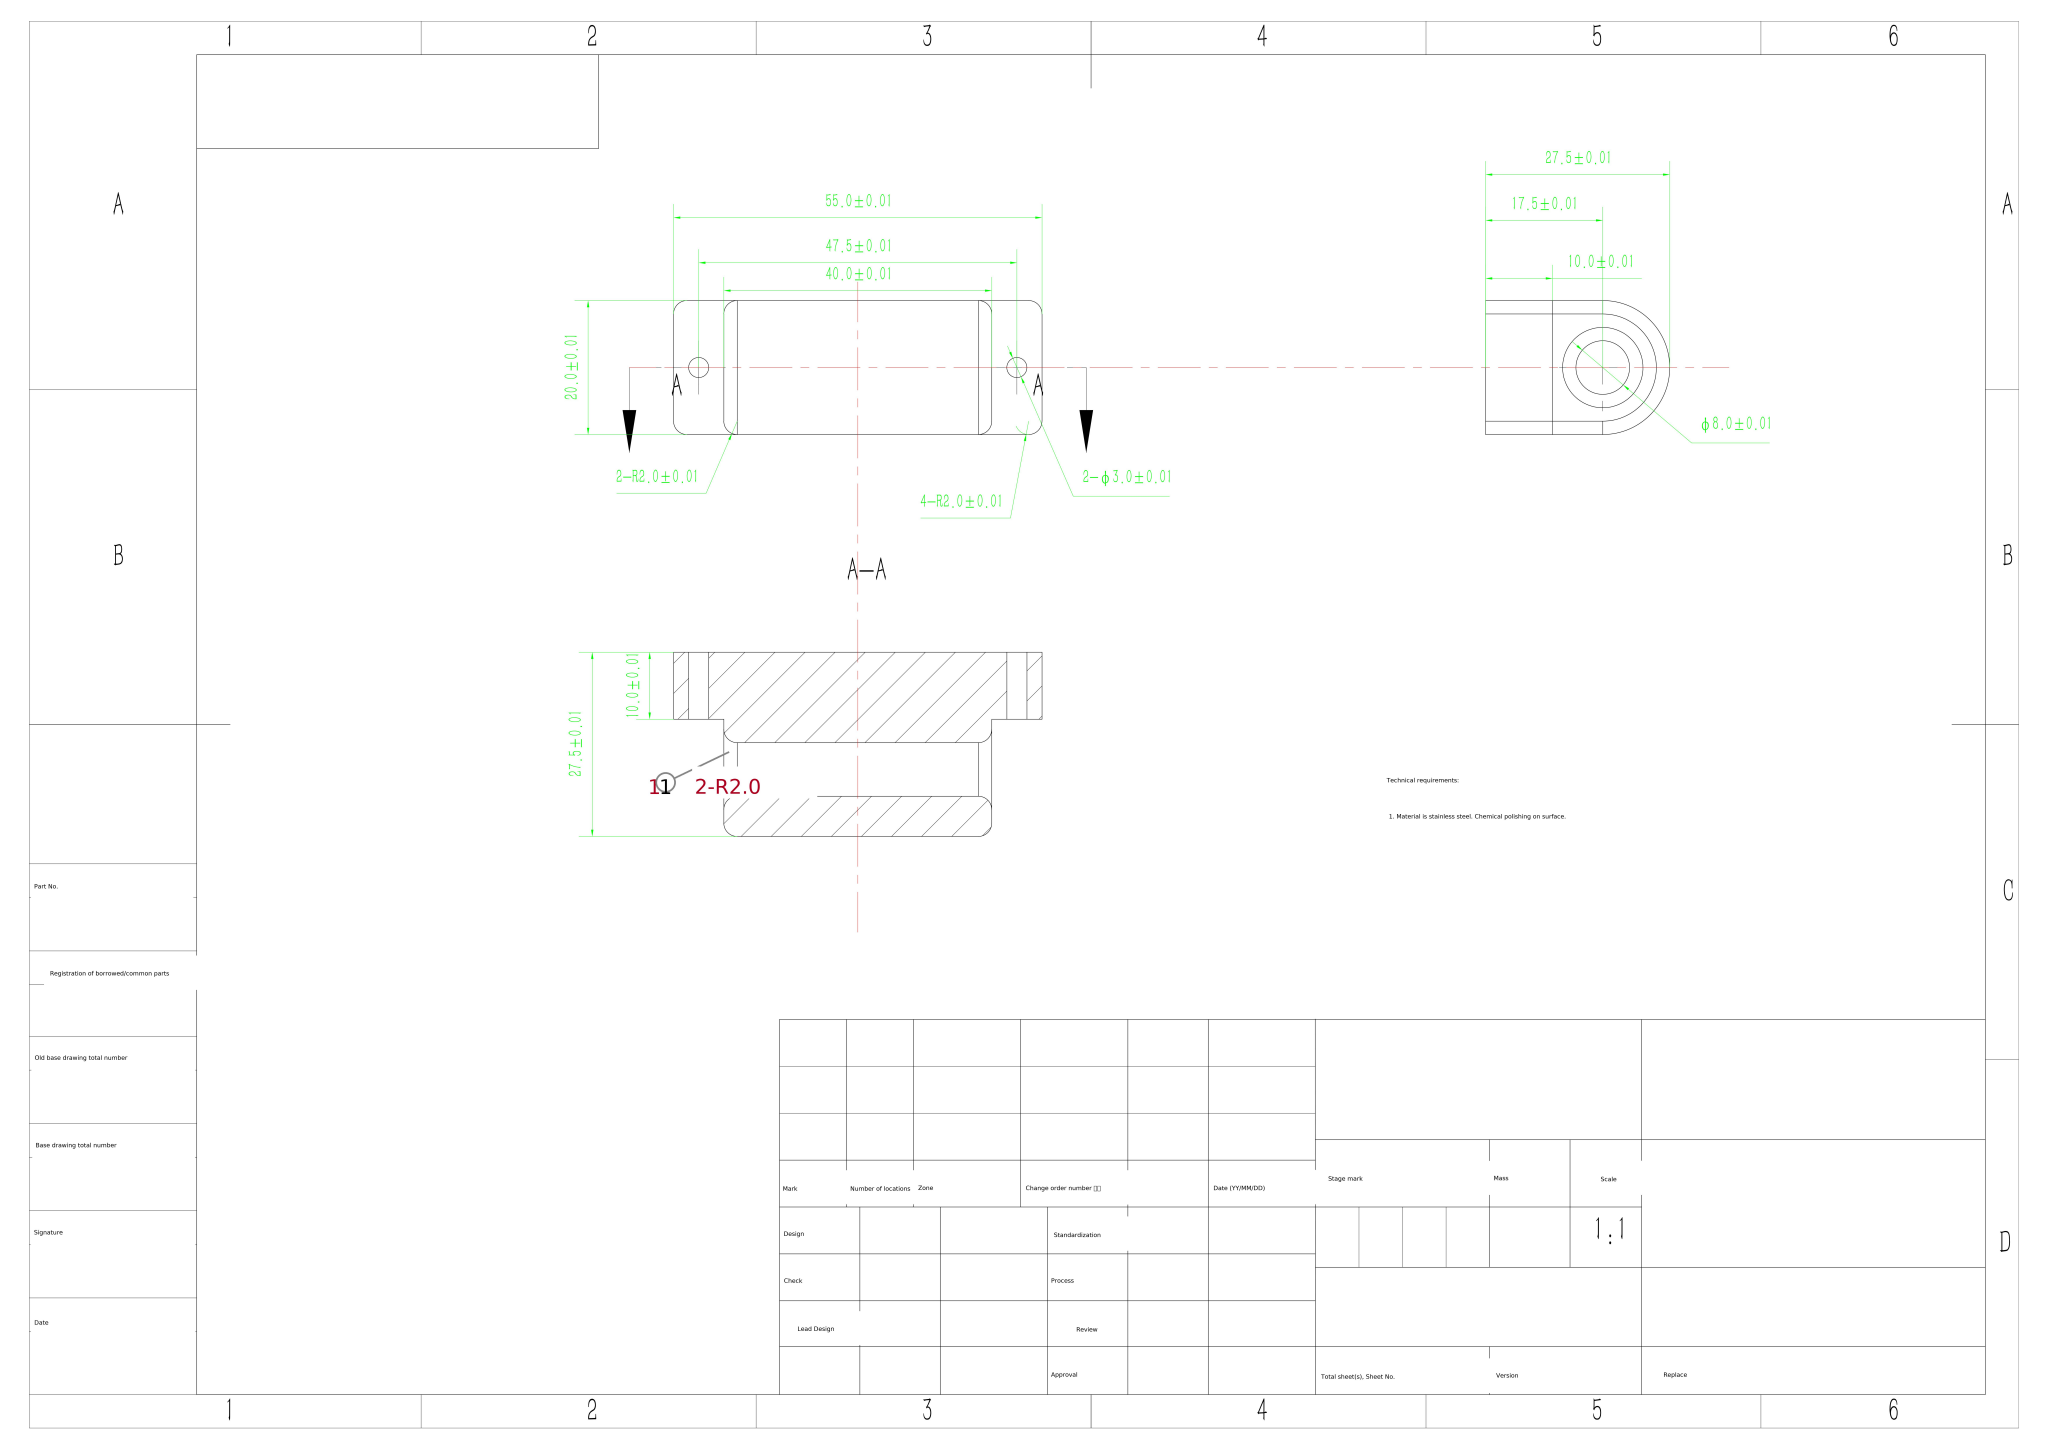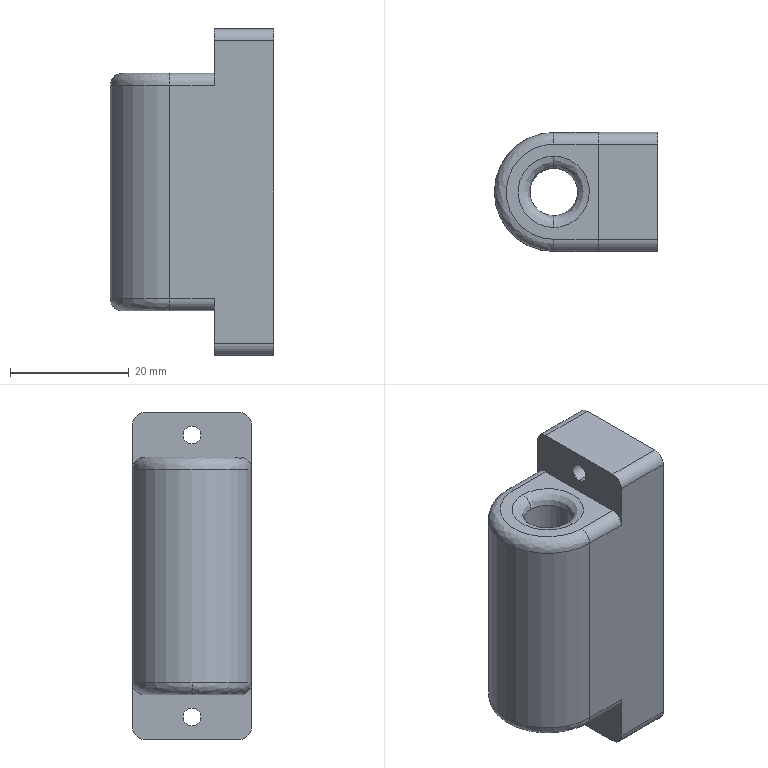Part | SolidWorks | mm | material stainless steel | 1 solid | 31 faces | box 27.5 x 20 x 55 mm | volume 20969 mm3 | cylinder 15 | plane 9 | spline 7 | commonest cylinder face diameters 4 x8 3 x4 8 x2 20 x1